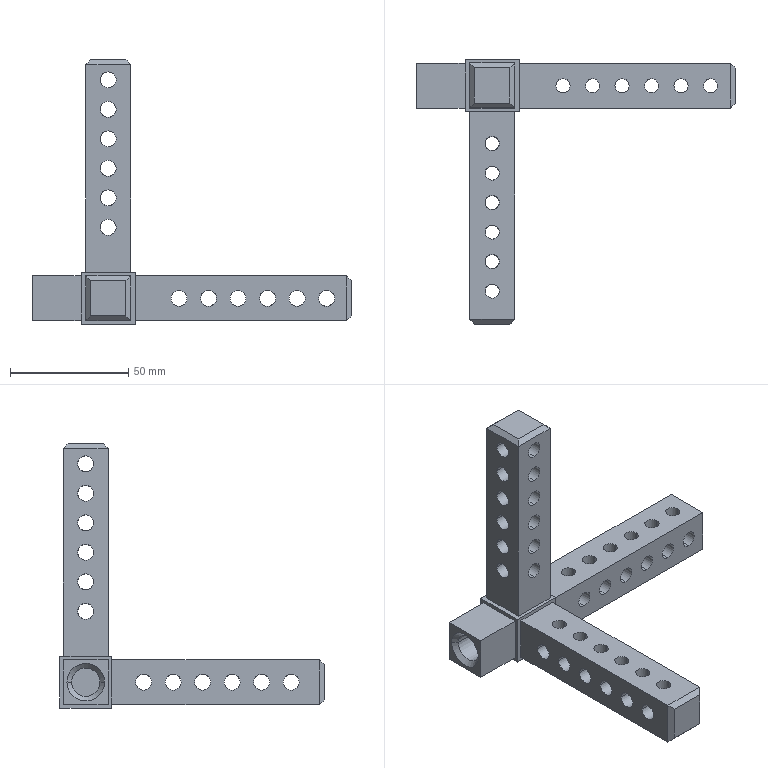Component | SolidWorks | CabinetFrameWeldmentDrawingPG50-01-00-1_FrameConnectionTee2(PG50-01-104-1 | 1 solid | 168 faces | box 135 x 112 x 112 mm | volume 94075 mm3 | cylinder 122 | plane 44 | cone 2 | commonest cylinder face diameters 6.8 x72 6 x48 12 x2 | material AISI 1045 Steel, cold drawn
build123d program:
from build123d import *

# Parameters (mm, degrees)
BOSS_EXTRUDE1_DEPTH      = 9.5
SKETCH2_W                = 19
SKETCH2_H                = 19
BOSS_EXTRUDE2_DEPTH      = 91.5
SKETCH3_W                = 19
SKETCH3_H                = 19
BOSS_EXTRUDE3_DEPTH      = 22.5
SKETCH4_R                = 6
CUT_EXTRUDE1_2_DEPTH     = 20
CHAMFER1_SIZE            = 2
BOSS_EXTRUDE4_DEPTH      = 1.5
BOSS_EXTRUDE4_DEPTH_BACK = 20.5
SKETCH5_W                = 22
SKETCH5_H                = 23
CHAMFER3_SIZE            = 2
SKETCH7_R                = 3.4
CUT_EXTRUDE2_DEPTH       = 183.315
SKETCH8_R                = 3.4
CUT_EXTRUDE3_DEPTH       = 188.263
SKETCH9_R                = 3
CUT_EXTRUDE4_DEPTH       = 188.263
SKETCH1_W                = 23
SKETCH1_H                = 23
SKETCH1_W_2              = 19.2
SKETCH1_H_2              = 19.2
CUT_EXTRUDE1_DEPTH       = 0.02


with BuildPart() as part:
    # Sketch1_2 → Boss-Extrude1 (new, symmetric)
    with BuildSketch(Plane.XY):
        Polygon((0, 0), (110.5, 0), (110.5, -19), (19, -19), (19, -112.5), (0, -112.5), align=None)
    extrude(amount=BOSS_EXTRUDE1_DEPTH, both=True)

    # Sketch2 → Boss-Extrude2 (add)
    with BuildSketch(Plane.XY.offset(9.5)):
        with Locations((9.5, -9.5)):
            Rectangle(SKETCH2_W, SKETCH2_H)
    extrude(amount=BOSS_EXTRUDE2_DEPTH)

    # Sketch3 → Boss-Extrude3 (add)
    with BuildSketch(Plane(origin=(0, 0, 0), x_dir=(1, 0, 0), z_dir=(0, 1, 0))):
        with Locations((9.5, 0)):
            Rectangle(SKETCH3_W, SKETCH3_H)
    extrude(amount=BOSS_EXTRUDE3_DEPTH)

    # Sketch4 → Cut-Extrude1_2 (cut)
    with BuildSketch(Plane(origin=(0, 22.5, 0), x_dir=(1, 0, 0), z_dir=(0, 1, 0))):
        with Locations(Location((9.5, 0, 0), (0, 0, 270))):
            Circle(SKETCH4_R)
    extrude(amount=-CUT_EXTRUDE1_2_DEPTH, mode=Mode.SUBTRACT)

    # Chamfer1
    chamfer1_edges = [part.edges().sort_by_distance(p)[0] for p in [
        (9.5, 22.5, -6),
    ]]
    chamfer(chamfer1_edges, length=CHAMFER1_SIZE)

    # Sketch5 → Boss-Extrude4 (add, two sides: drawn at the far end of the back side and taken through both)
    with BuildSketch(Plane.XY.offset(9.5).offset(-BOSS_EXTRUDE4_DEPTH_BACK)):
        with Locations((9.5, -9.5)):
            Rectangle(SKETCH5_W, SKETCH5_H)
    extrude(amount=BOSS_EXTRUDE4_DEPTH + BOSS_EXTRUDE4_DEPTH_BACK)

    # Chamfer3
    chamfer3_edges = [part.edges().sort_by_distance(p)[0] for p in [
        (110.5, 0, 0),
        (110.5, -19, 0),
        (19, -112.5, 0),
        (0, -112.5, 0),
        (110.5, -9.5, 9.5),
        (0, -9.5, 101),
        (9.5, -19, 101),
        (19, -9.5, 101),
        (9.5, 0, 101),
        (110.5, -9.5, -9.5),
        (9.5, -112.5, 9.5),
        (9.5, -112.5, -9.5),
    ]]
    chamfer(chamfer3_edges, length=CHAMFER3_SIZE)

    # Sketch7 → Cut-Extrude2 (cut, through all)
    with BuildSketch(Plane.XY.offset(9.5)):
        with Locations((102, -9.5)):
            Circle(SKETCH7_R)
        with Locations((89.5, -9.5)):
            Circle(SKETCH7_R)
        with Locations((77, -9.5)):
            Circle(SKETCH7_R)
        with Locations((64.5, -9.5)):
            Circle(SKETCH7_R)
        with Locations((52, -9.5)):
            Circle(SKETCH7_R)
        with Locations((39.5, -9.5)):
            Circle(SKETCH7_R)
        with Locations((9.5, -102)):
            Circle(SKETCH7_R)
        with Locations((9.5, -89.5)):
            Circle(SKETCH7_R)
        with Locations((9.5, -77)):
            Circle(SKETCH7_R)
        with Locations((9.5, -64.5)):
            Circle(SKETCH7_R)
        with Locations((9.5, -52)):
            Circle(SKETCH7_R)
        with Locations((9.5, -39.5)):
            Circle(SKETCH7_R)
    extrude(amount=-CUT_EXTRUDE2_DEPTH, mode=Mode.SUBTRACT)

    # Sketch8 → Cut-Extrude3 (cut, through all)
    with BuildSketch(Plane(origin=(0, 0, 0), x_dir=(1, 0, 0), z_dir=(0, 1, 0))):
        with Locations(Location((9.5, -87, 0), (0, 0, 270))):
            Circle(SKETCH8_R)
        with Locations(Location((9.5, -74.5, 0), (0, 0, 270))):
            Circle(SKETCH8_R)
        with Locations(Location((9.5, -62, 0), (0, 0, 270))):
            Circle(SKETCH8_R)
        with Locations(Location((9.5, -49.5, 0), (0, 0, 270))):
            Circle(SKETCH8_R)
        with Locations(Location((9.5, -37, 0), (0, 0, 270))):
            Circle(SKETCH8_R)
        with Locations(Location((102, 0, 0), (0, 0, 270))):
            Circle(SKETCH8_R)
        with Locations(Location((89.5, 0, 0), (0, 0, 270))):
            Circle(SKETCH8_R)
        with Locations(Location((77, 0, 0), (0, 0, 270))):
            Circle(SKETCH8_R)
        with Locations(Location((64.5, 0, 0), (0, 0, 270))):
            Circle(SKETCH8_R)
        with Locations(Location((52, 0, 0), (0, 0, 270))):
            Circle(SKETCH8_R)
        with Locations(Location((39.5, 0, 0), (0, 0, 270))):
            Circle(SKETCH8_R)
        with Locations(Location((9.5, -24.5, 0), (0, 0, 270))):
            Circle(SKETCH8_R)
    extrude(amount=-CUT_EXTRUDE3_DEPTH, mode=Mode.SUBTRACT)

    # Sketch9 → Cut-Extrude4 (cut, through all)
    with BuildSketch(Plane.ZY):
        with Locations(Location((24.5, -9.5, 0), (0, 0, 270))):
            Circle(SKETCH9_R)
        with Locations(Location((37, -9.5, 0), (0, 0, 270))):
            Circle(SKETCH9_R)
        with Locations(Location((49.5, -9.5, 0), (0, 0, 270))):
            Circle(SKETCH9_R)
        with Locations(Location((62, -9.5, 0), (0, 0, 270))):
            Circle(SKETCH9_R)
        with Locations(Location((74.5, -9.5, 0), (0, 0, 270))):
            Circle(SKETCH9_R)
        with Locations(Location((87, -9.5, 0), (0, 0, 270))):
            Circle(SKETCH9_R)
        with Locations(Location((0, -39.5, 0), (0, 0, 270))):
            Circle(SKETCH9_R)
        with Locations(Location((0, -52, 0), (0, 0, 270))):
            Circle(SKETCH9_R)
        with Locations(Location((0, -64.5, 0), (0, 0, 270))):
            Circle(SKETCH9_R)
        with Locations(Location((0, -77, 0), (0, 0, 270))):
            Circle(SKETCH9_R)
        with Locations(Location((0, -89.5, 0), (0, 0, 270))):
            Circle(SKETCH9_R)
        with Locations(Location((0, -102, 0), (0, 0, 270))):
            Circle(SKETCH9_R)
    extrude(amount=-CUT_EXTRUDE4_DEPTH, mode=Mode.SUBTRACT)

    # Sketch1 → Cut-Extrude1 (cut)
    with BuildSketch(Plane.XZ.offset(21)):
        with Locations((9.5, 0)):
            Rectangle(SKETCH1_W, SKETCH1_H)
        with Locations((9.5, 0)):
            Rectangle(SKETCH1_W_2, SKETCH1_H_2, mode=Mode.SUBTRACT)
    extrude(amount=-CUT_EXTRUDE1_DEPTH, mode=Mode.SUBTRACT)


solid = part.part

# Placed as in the assembly
solid = solid.moved(Location((-1150.67, 277.207, -377.003), (90, 0, 90)))